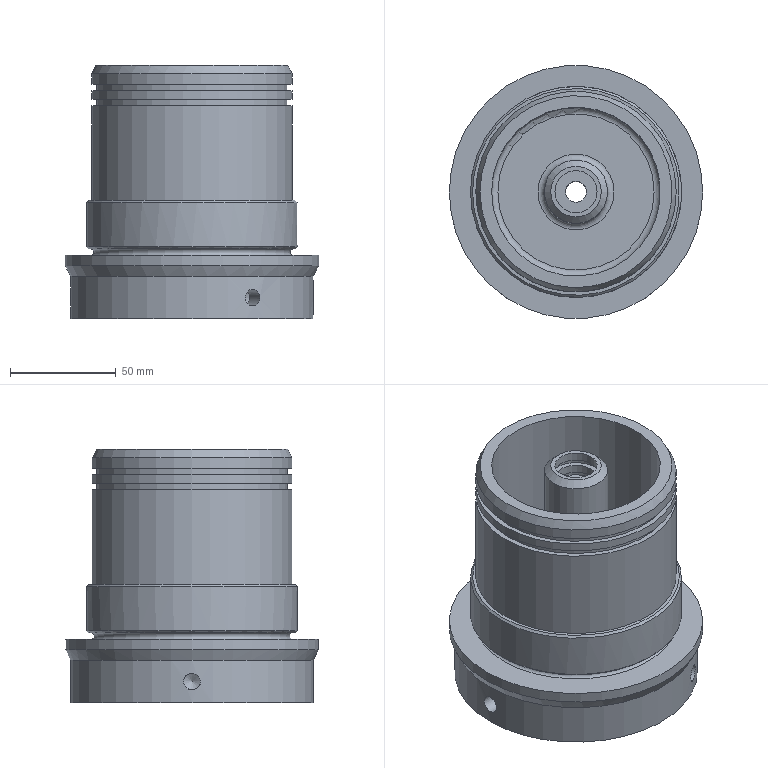Component | NX | CH3404_8-1 | 1 solid | 48 faces | volume 540780 mm3 | cylinder 20 | plane 16 | cone 9 | torus 3 | commonest cylinder face diameters 20 x3 95 x3 8 x3 24.6 x2 90.4 x2 120 x1 115 x1 10 x1